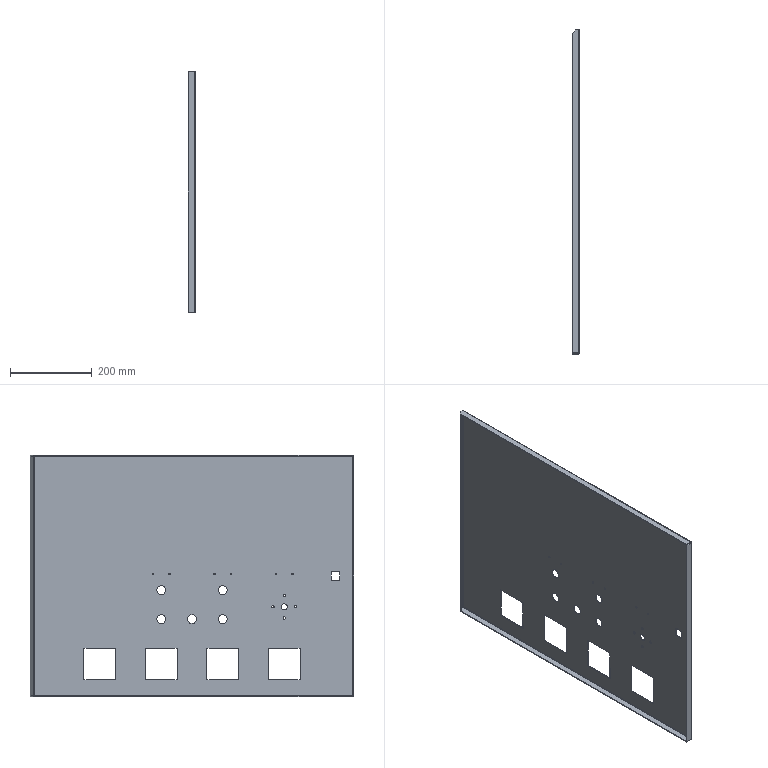Component | SolidWorks | FrontMiddleUpperDoor-1_FrontMiddleUpperDoor-1 | 1 solid | 111 faces | volume 965511 mm3 | plane 61 | cylinder 46 | spline 4 | commonest cylinder face diameters 6 x17 4 x12 22 x10 2 x5 15 x2